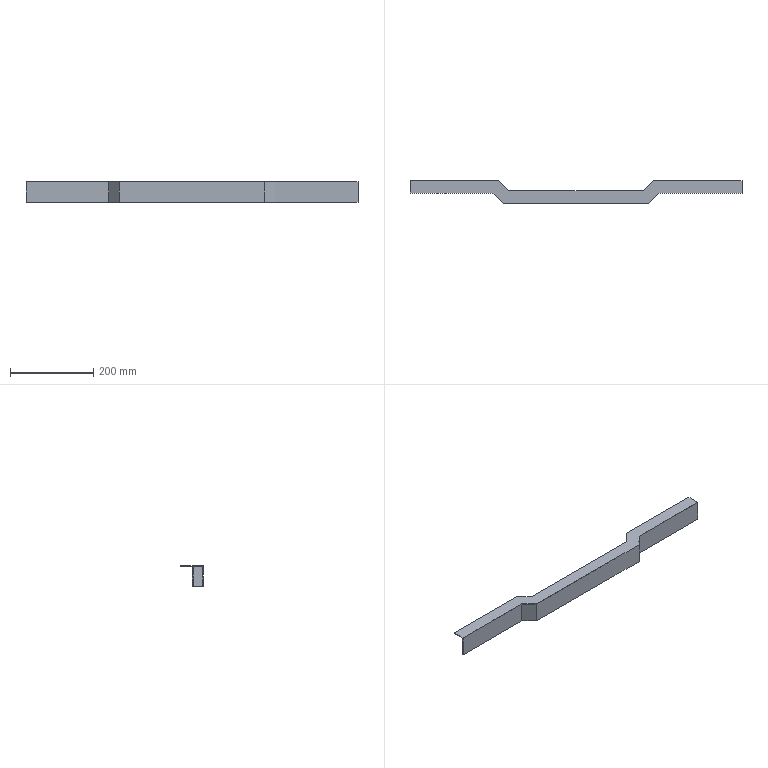Component | SolidWorks | JF21-80.1-1-3(_)-1-SOLID70-1 | 1 solid | 20 faces | box 800 x 55 x 50 mm | volume 128031 mm3 | plane 20
STEP:
#1=CARTESIAN_POINT('',(15.748,-7.677,-5.197));
#2=VERTEX_POINT('',#1);
#3=CARTESIAN_POINT('',(15.748,-7.677,-5.118));
#4=VERTEX_POINT('',#3);
#5=CARTESIAN_POINT('',(15.748,-7.677,-5.118));
#6=DIRECTION('',(0.,0.,1.));
#7=VECTOR('',#6,39.37);
#8=LINE('',#5,#7);
#9=EDGE_CURVE('',#2,#4,#8,.T.);
#10=ORIENTED_EDGE('',*,*,#9,.F.);
#11=CARTESIAN_POINT('',(7.385,-7.677,-5.197));
#12=VERTEX_POINT('',#11);
#13=CARTESIAN_POINT('',(7.385,-7.677,-5.197));
#14=DIRECTION('',(1.,-0.,0.));
#15=VECTOR('',#14,39.37);
#16=LINE('',#13,#15);
#17=EDGE_CURVE('',#12,#2,#16,.T.);
#18=ORIENTED_EDGE('',*,*,#17,.F.);
#19=CARTESIAN_POINT('',(7.385,-7.677,-5.118));
#20=VERTEX_POINT('',#19);
#21=CARTESIAN_POINT('',(7.385,-7.677,-5.118));
#22=DIRECTION('',(0.,0.,-1.));
#23=VECTOR('',#22,39.37);
#24=LINE('',#21,#23);
#25=EDGE_CURVE('',#20,#12,#24,.T.);
#26=ORIENTED_EDGE('',*,*,#25,.F.);
#27=CARTESIAN_POINT('',(7.385,-7.677,-5.118));
#28=DIRECTION('',(1.,-0.,0.));
#29=VECTOR('',#28,39.37);
#30=LINE('',#27,#29);
#31=EDGE_CURVE('',#20,#4,#30,.T.);
#32=ORIENTED_EDGE('',*,*,#31,.T.);
#33=EDGE_LOOP('',(#10,#18,#26,#32));
#34=FACE_OUTER_BOUND('',#33,.T.);
#35=CARTESIAN_POINT('',(7.385,-7.677,-5.118));
#36=DIRECTION('',(-0.,-1.,0.));
#37=DIRECTION('',(-1.,0.,0.));
#38=AXIS2_PLACEMENT_3D('',#35,#36,#37);
#39=PLANE('',#38);
#40=ADVANCED_FACE('',(#34),#39,.F.);
#41=CARTESIAN_POINT('',(15.748,-8.78,-7.087));
#42=VERTEX_POINT('',#41);
#43=CARTESIAN_POINT('',(15.748,-8.78,-5.197));
#44=VERTEX_POINT('',#43);
#45=CARTESIAN_POINT('',(15.748,-8.78,-5.197));
#46=DIRECTION('',(0.,0.,1.));
#47=VECTOR('',#46,39.37);
#48=LINE('',#45,#47);
#49=EDGE_CURVE('',#42,#44,#48,.T.);
#50=ORIENTED_EDGE('',*,*,#49,.F.);
#51=CARTESIAN_POINT('',(7.841,-8.78,-7.087));
#52=VERTEX_POINT('',#51);
#53=CARTESIAN_POINT('',(7.841,-8.78,-7.087));
#54=DIRECTION('',(1.,-0.,0.));
#55=VECTOR('',#54,39.37);
#56=LINE('',#53,#55);
#57=EDGE_CURVE('',#52,#42,#56,.T.);
#58=ORIENTED_EDGE('',*,*,#57,.F.);
#59=CARTESIAN_POINT('',(7.841,-8.78,-5.197));
#60=VERTEX_POINT('',#59);
#61=CARTESIAN_POINT('',(7.841,-8.78,-5.197));
#62=DIRECTION('',(0.,0.,-1.));
#63=VECTOR('',#62,39.37);
#64=LINE('',#61,#63);
#65=EDGE_CURVE('',#60,#52,#64,.T.);
#66=ORIENTED_EDGE('',*,*,#65,.F.);
#67=CARTESIAN_POINT('',(7.841,-8.78,-5.197));
#68=DIRECTION('',(1.,-0.,0.));
#69=VECTOR('',#68,39.37);
#70=LINE('',#67,#69);
#71=EDGE_CURVE('',#60,#44,#70,.T.);
#72=ORIENTED_EDGE('',*,*,#71,.T.);
#73=EDGE_LOOP('',(#50,#58,#66,#72));
#74=FACE_OUTER_BOUND('',#73,.T.);
#75=CARTESIAN_POINT('',(7.841,-8.78,-5.197));
#76=DIRECTION('',(-0.,-1.,0.));
#77=DIRECTION('',(-1.,0.,0.));
#78=AXIS2_PLACEMENT_3D('',#75,#76,#77);
#79=PLANE('',#78);
#80=ADVANCED_FACE('',(#74),#79,.F.);
#81=CARTESIAN_POINT('',(15.748,-8.858,-5.118));
#82=VERTEX_POINT('',#81);
#83=CARTESIAN_POINT('',(15.748,-8.858,-7.087));
#84=VERTEX_POINT('',#83);
#85=CARTESIAN_POINT('',(15.748,-8.858,-7.087));
#86=DIRECTION('',(0.,0.,-1.));
#87=VECTOR('',#86,39.37);
#88=LINE('',#85,#87);
#89=EDGE_CURVE('',#82,#84,#88,.T.);
#90=ORIENTED_EDGE('',*,*,#89,.F.);
#91=CARTESIAN_POINT('',(7.874,-8.858,-5.118));
#92=VERTEX_POINT('',#91);
#93=CARTESIAN_POINT('',(7.874,-8.858,-5.118));
#94=DIRECTION('',(1.,-0.,0.));
#95=VECTOR('',#94,39.37);
#96=LINE('',#93,#95);
#97=EDGE_CURVE('',#92,#82,#96,.T.);
#98=ORIENTED_EDGE('',*,*,#97,.F.);
#99=CARTESIAN_POINT('',(7.874,-8.858,-7.087));
#100=VERTEX_POINT('',#99);
#101=CARTESIAN_POINT('',(7.874,-8.858,-7.087));
#102=DIRECTION('',(0.,0.,1.));
#103=VECTOR('',#102,39.37);
#104=LINE('',#101,#103);
#105=EDGE_CURVE('',#100,#92,#104,.T.);
#106=ORIENTED_EDGE('',*,*,#105,.F.);
#107=CARTESIAN_POINT('',(7.874,-8.858,-7.087));
#108=DIRECTION('',(1.,-0.,0.));
#109=VECTOR('',#108,39.37);
#110=LINE('',#107,#109);
#111=EDGE_CURVE('',#100,#84,#110,.T.);
#112=ORIENTED_EDGE('',*,*,#111,.T.);
#113=EDGE_LOOP('',(#90,#98,#106,#112));
#114=FACE_OUTER_BOUND('',#113,.T.);
#115=CARTESIAN_POINT('',(7.874,-8.858,-7.087));
#116=DIRECTION('',(0.,1.,0.));
#117=DIRECTION('',(1.,-0.,0.));
#118=AXIS2_PLACEMENT_3D('',#115,#116,#117);
#119=PLANE('',#118);
#120=ADVANCED_FACE('',(#114),#119,.F.);
#121=CARTESIAN_POINT('',(6.857,-9.764,-5.197));
#122=VERTEX_POINT('',#121);
#123=CARTESIAN_POINT('',(6.857,-9.764,-5.197));
#124=DIRECTION('',(0.7071,0.7071,0.));
#125=VECTOR('',#124,39.37);
#126=LINE('',#123,#125);
#127=EDGE_CURVE('',#122,#60,#126,.T.);
#128=ORIENTED_EDGE('',*,*,#127,.T.);
#129=ORIENTED_EDGE('',*,*,#65,.T.);
#130=CARTESIAN_POINT('',(6.857,-9.764,-7.087));
#131=VERTEX_POINT('',#130);
#132=CARTESIAN_POINT('',(6.857,-9.764,-7.087));
#133=DIRECTION('',(0.7071,0.7071,0.));
#134=VECTOR('',#133,39.37);
#135=LINE('',#132,#134);
#136=EDGE_CURVE('',#131,#52,#135,.T.);
#137=ORIENTED_EDGE('',*,*,#136,.F.);
#138=CARTESIAN_POINT('',(6.857,-9.764,-5.197));
#139=DIRECTION('',(0.,0.,1.));
#140=VECTOR('',#139,39.37);
#141=LINE('',#138,#140);
#142=EDGE_CURVE('',#131,#122,#141,.T.);
#143=ORIENTED_EDGE('',*,*,#142,.T.);
#144=EDGE_LOOP('',(#128,#129,#137,#143));
#145=FACE_OUTER_BOUND('',#144,.T.);
#146=CARTESIAN_POINT('',(6.857,-9.764,-5.197));
#147=DIRECTION('',(-0.7071,0.7071,0.));
#148=DIRECTION('',(0.7071,0.7071,0.));
#149=AXIS2_PLACEMENT_3D('',#146,#147,#148);
#150=PLANE('',#149);
#151=ADVANCED_FACE('',(#145),#150,.T.);
#152=CARTESIAN_POINT('',(6.89,-9.843,-7.087));
#153=VERTEX_POINT('',#152);
#154=CARTESIAN_POINT('',(6.89,-9.843,-7.087));
#155=DIRECTION('',(0.7071,0.7071,0.));
#156=VECTOR('',#155,39.37);
#157=LINE('',#154,#156);
#158=EDGE_CURVE('',#153,#100,#157,.T.);
#159=ORIENTED_EDGE('',*,*,#158,.T.);
#160=ORIENTED_EDGE('',*,*,#105,.T.);
#161=CARTESIAN_POINT('',(6.89,-9.843,-5.118));
#162=VERTEX_POINT('',#161);
#163=CARTESIAN_POINT('',(6.89,-9.843,-5.118));
#164=DIRECTION('',(0.7071,0.7071,0.));
#165=VECTOR('',#164,39.37);
#166=LINE('',#163,#165);
#167=EDGE_CURVE('',#162,#92,#166,.T.);
#168=ORIENTED_EDGE('',*,*,#167,.F.);
#169=CARTESIAN_POINT('',(6.89,-9.843,-7.087));
#170=DIRECTION('',(0.,0.,-1.));
#171=VECTOR('',#170,39.37);
#172=LINE('',#169,#171);
#173=EDGE_CURVE('',#162,#153,#172,.T.);
#174=ORIENTED_EDGE('',*,*,#173,.T.);
#175=EDGE_LOOP('',(#159,#160,#168,#174));
#176=FACE_OUTER_BOUND('',#175,.T.);
#177=CARTESIAN_POINT('',(6.89,-9.843,-7.087));
#178=DIRECTION('',(0.7071,-0.7071,0.));
#179=DIRECTION('',(-0.7071,-0.7071,0.));
#180=AXIS2_PLACEMENT_3D('',#177,#178,#179);
#181=PLANE('',#180);
#182=ADVANCED_FACE('',(#176),#181,.T.);
#183=CARTESIAN_POINT('',(6.401,-8.661,-5.118));
#184=VERTEX_POINT('',#183);
#185=CARTESIAN_POINT('',(6.401,-8.661,-5.118));
#186=DIRECTION('',(0.7071,0.7071,0.));
#187=VECTOR('',#186,39.37);
#188=LINE('',#185,#187);
#189=EDGE_CURVE('',#184,#20,#188,.T.);
#190=ORIENTED_EDGE('',*,*,#189,.T.);
#191=ORIENTED_EDGE('',*,*,#25,.T.);
#192=CARTESIAN_POINT('',(6.401,-8.661,-5.197));
#193=VERTEX_POINT('',#192);
#194=CARTESIAN_POINT('',(6.401,-8.661,-5.197));
#195=DIRECTION('',(0.7071,0.7071,0.));
#196=VECTOR('',#195,39.37);
#197=LINE('',#194,#196);
#198=EDGE_CURVE('',#193,#12,#197,.T.);
#199=ORIENTED_EDGE('',*,*,#198,.F.);
#200=CARTESIAN_POINT('',(6.401,-8.661,-5.118));
#201=DIRECTION('',(0.,0.,1.));
#202=VECTOR('',#201,39.37);
#203=LINE('',#200,#202);
#204=EDGE_CURVE('',#193,#184,#203,.T.);
#205=ORIENTED_EDGE('',*,*,#204,.T.);
#206=EDGE_LOOP('',(#190,#191,#199,#205));
#207=FACE_OUTER_BOUND('',#206,.T.);
#208=CARTESIAN_POINT('',(6.401,-8.661,-5.118));
#209=DIRECTION('',(-0.7071,0.7071,0.));
#210=DIRECTION('',(0.7071,0.7071,0.));
#211=AXIS2_PLACEMENT_3D('',#208,#209,#210);
#212=PLANE('',#211);
#213=ADVANCED_FACE('',(#207),#212,.T.);
#214=ORIENTED_EDGE('',*,*,#142,.F.);
#215=CARTESIAN_POINT('',(-6.857,-9.764,-7.087));
#216=VERTEX_POINT('',#215);
#217=CARTESIAN_POINT('',(-6.857,-9.764,-7.087));
#218=DIRECTION('',(1.,-0.,0.));
#219=VECTOR('',#218,39.37);
#220=LINE('',#217,#219);
#221=EDGE_CURVE('',#216,#131,#220,.T.);
#222=ORIENTED_EDGE('',*,*,#221,.F.);
#223=CARTESIAN_POINT('',(-6.857,-9.764,-5.197));
#224=VERTEX_POINT('',#223);
#225=CARTESIAN_POINT('',(-6.857,-9.764,-5.197));
#226=DIRECTION('',(0.,0.,-1.));
#227=VECTOR('',#226,39.37);
#228=LINE('',#225,#227);
#229=EDGE_CURVE('',#224,#216,#228,.T.);
#230=ORIENTED_EDGE('',*,*,#229,.F.);
#231=CARTESIAN_POINT('',(-6.857,-9.764,-5.197));
#232=DIRECTION('',(1.,-0.,0.));
#233=VECTOR('',#232,39.37);
#234=LINE('',#231,#233);
#235=EDGE_CURVE('',#224,#122,#234,.T.);
#236=ORIENTED_EDGE('',*,*,#235,.T.);
#237=EDGE_LOOP('',(#214,#222,#230,#236));
#238=FACE_OUTER_BOUND('',#237,.T.);
#239=CARTESIAN_POINT('',(-6.857,-9.764,-5.197));
#240=DIRECTION('',(-0.,-1.,0.));
#241=DIRECTION('',(-1.,0.,0.));
#242=AXIS2_PLACEMENT_3D('',#239,#240,#241);
#243=PLANE('',#242);
#244=ADVANCED_FACE('',(#238),#243,.F.);
#245=ORIENTED_EDGE('',*,*,#173,.F.);
#246=CARTESIAN_POINT('',(-6.89,-9.843,-5.118));
#247=VERTEX_POINT('',#246);
#248=CARTESIAN_POINT('',(-6.89,-9.843,-5.118));
#249=DIRECTION('',(1.,-0.,0.));
#250=VECTOR('',#249,39.37);
#251=LINE('',#248,#250);
#252=EDGE_CURVE('',#247,#162,#251,.T.);
#253=ORIENTED_EDGE('',*,*,#252,.F.);
#254=CARTESIAN_POINT('',(-6.89,-9.843,-7.087));
#255=VERTEX_POINT('',#254);
#256=CARTESIAN_POINT('',(-6.89,-9.843,-7.087));
#257=DIRECTION('',(0.,0.,1.));
#258=VECTOR('',#257,39.37);
#259=LINE('',#256,#258);
#260=EDGE_CURVE('',#255,#247,#259,.T.);
#261=ORIENTED_EDGE('',*,*,#260,.F.);
#262=CARTESIAN_POINT('',(-6.89,-9.843,-7.087));
#263=DIRECTION('',(1.,-0.,0.));
#264=VECTOR('',#263,39.37);
#265=LINE('',#262,#264);
#266=EDGE_CURVE('',#255,#153,#265,.T.);
#267=ORIENTED_EDGE('',*,*,#266,.T.);
#268=EDGE_LOOP('',(#245,#253,#261,#267));
#269=FACE_OUTER_BOUND('',#268,.T.);
#270=CARTESIAN_POINT('',(-6.89,-9.843,-7.087));
#271=DIRECTION('',(0.,1.,0.));
#272=DIRECTION('',(1.,-0.,0.));
#273=AXIS2_PLACEMENT_3D('',#270,#271,#272);
#274=PLANE('',#273);
#275=ADVANCED_FACE('',(#269),#274,.F.);
#276=ORIENTED_EDGE('',*,*,#204,.F.);
#277=CARTESIAN_POINT('',(-6.401,-8.661,-5.197));
#278=VERTEX_POINT('',#277);
#279=CARTESIAN_POINT('',(-6.401,-8.661,-5.197));
#280=DIRECTION('',(1.,-0.,0.));
#281=VECTOR('',#280,39.37);
#282=LINE('',#279,#281);
#283=EDGE_CURVE('',#278,#193,#282,.T.);
#284=ORIENTED_EDGE('',*,*,#283,.F.);
#285=CARTESIAN_POINT('',(-6.401,-8.661,-5.118));
#286=VERTEX_POINT('',#285);
#287=CARTESIAN_POINT('',(-6.401,-8.661,-5.118));
#288=DIRECTION('',(0.,0.,-1.));
#289=VECTOR('',#288,39.37);
#290=LINE('',#287,#289);
#291=EDGE_CURVE('',#286,#278,#290,.T.);
#292=ORIENTED_EDGE('',*,*,#291,.F.);
#293=CARTESIAN_POINT('',(-6.401,-8.661,-5.118));
#294=DIRECTION('',(1.,-0.,0.));
#295=VECTOR('',#294,39.37);
#296=LINE('',#293,#295);
#297=EDGE_CURVE('',#286,#184,#296,.T.);
#298=ORIENTED_EDGE('',*,*,#297,.T.);
#299=EDGE_LOOP('',(#276,#284,#292,#298));
#300=FACE_OUTER_BOUND('',#299,.T.);
#301=CARTESIAN_POINT('',(-6.401,-8.661,-5.118));
#302=DIRECTION('',(-0.,-1.,0.));
#303=DIRECTION('',(-1.,0.,0.));
#304=AXIS2_PLACEMENT_3D('',#301,#302,#303);
#305=PLANE('',#304);
#306=ADVANCED_FACE('',(#300),#305,.F.);
#307=CARTESIAN_POINT('',(-7.841,-8.78,-5.197));
#308=VERTEX_POINT('',#307);
#309=CARTESIAN_POINT('',(-7.841,-8.78,-5.197));
#310=DIRECTION('',(0.7071,-0.7071,0.));
#311=VECTOR('',#310,39.37);
#312=LINE('',#309,#311);
#313=EDGE_CURVE('',#308,#224,#312,.T.);
#314=ORIENTED_EDGE('',*,*,#313,.T.);
#315=ORIENTED_EDGE('',*,*,#229,.T.);
#316=CARTESIAN_POINT('',(-7.841,-8.78,-7.087));
#317=VERTEX_POINT('',#316);
#318=CARTESIAN_POINT('',(-7.841,-8.78,-7.087));
#319=DIRECTION('',(0.7071,-0.7071,0.));
#320=VECTOR('',#319,39.37);
#321=LINE('',#318,#320);
#322=EDGE_CURVE('',#317,#216,#321,.T.);
#323=ORIENTED_EDGE('',*,*,#322,.F.);
#324=CARTESIAN_POINT('',(-7.841,-8.78,-5.197));
#325=DIRECTION('',(0.,0.,1.));
#326=VECTOR('',#325,39.37);
#327=LINE('',#324,#326);
#328=EDGE_CURVE('',#317,#308,#327,.T.);
#329=ORIENTED_EDGE('',*,*,#328,.T.);
#330=EDGE_LOOP('',(#314,#315,#323,#329));
#331=FACE_OUTER_BOUND('',#330,.T.);
#332=CARTESIAN_POINT('',(-7.841,-8.78,-5.197));
#333=DIRECTION('',(0.7071,0.7071,0.));
#334=DIRECTION('',(0.7071,-0.7071,0.));
#335=AXIS2_PLACEMENT_3D('',#332,#333,#334);
#336=PLANE('',#335);
#337=ADVANCED_FACE('',(#331),#336,.T.);
#338=CARTESIAN_POINT('',(-7.874,-8.858,-7.087));
#339=VERTEX_POINT('',#338);
#340=CARTESIAN_POINT('',(-7.874,-8.858,-7.087));
#341=DIRECTION('',(0.7071,-0.7071,0.));
#342=VECTOR('',#341,39.37);
#343=LINE('',#340,#342);
#344=EDGE_CURVE('',#339,#255,#343,.T.);
#345=ORIENTED_EDGE('',*,*,#344,.T.);
#346=ORIENTED_EDGE('',*,*,#260,.T.);
#347=CARTESIAN_POINT('',(-7.874,-8.858,-5.118));
#348=VERTEX_POINT('',#347);
#349=CARTESIAN_POINT('',(-7.874,-8.858,-5.118));
#350=DIRECTION('',(0.7071,-0.7071,0.));
#351=VECTOR('',#350,39.37);
#352=LINE('',#349,#351);
#353=EDGE_CURVE('',#348,#247,#352,.T.);
#354=ORIENTED_EDGE('',*,*,#353,.F.);
#355=CARTESIAN_POINT('',(-7.874,-8.858,-7.087));
#356=DIRECTION('',(0.,0.,-1.));
#357=VECTOR('',#356,39.37);
#358=LINE('',#355,#357);
#359=EDGE_CURVE('',#348,#339,#358,.T.);
#360=ORIENTED_EDGE('',*,*,#359,.T.);
#361=EDGE_LOOP('',(#345,#346,#354,#360));
#362=FACE_OUTER_BOUND('',#361,.T.);
#363=CARTESIAN_POINT('',(-7.874,-8.858,-7.087));
#364=DIRECTION('',(-0.7071,-0.7071,0.));
#365=DIRECTION('',(-0.7071,0.7071,0.));
#366=AXIS2_PLACEMENT_3D('',#363,#364,#365);
#367=PLANE('',#366);
#368=ADVANCED_FACE('',(#362),#367,.T.);
#369=CARTESIAN_POINT('',(-7.385,-7.677,-5.118));
#370=VERTEX_POINT('',#369);
#371=CARTESIAN_POINT('',(-7.385,-7.677,-5.118));
#372=DIRECTION('',(0.7071,-0.7071,0.));
#373=VECTOR('',#372,39.37);
#374=LINE('',#371,#373);
#375=EDGE_CURVE('',#370,#286,#374,.T.);
#376=ORIENTED_EDGE('',*,*,#375,.T.);
#377=ORIENTED_EDGE('',*,*,#291,.T.);
#378=CARTESIAN_POINT('',(-7.385,-7.677,-5.197));
#379=VERTEX_POINT('',#378);
#380=CARTESIAN_POINT('',(-7.385,-7.677,-5.197));
#381=DIRECTION('',(0.7071,-0.7071,0.));
#382=VECTOR('',#381,39.37);
#383=LINE('',#380,#382);
#384=EDGE_CURVE('',#379,#278,#383,.T.);
#385=ORIENTED_EDGE('',*,*,#384,.F.);
#386=CARTESIAN_POINT('',(-7.385,-7.677,-5.118));
#387=DIRECTION('',(0.,0.,1.));
#388=VECTOR('',#387,39.37);
#389=LINE('',#386,#388);
#390=EDGE_CURVE('',#379,#370,#389,.T.);
#391=ORIENTED_EDGE('',*,*,#390,.T.);
#392=EDGE_LOOP('',(#376,#377,#385,#391));
#393=FACE_OUTER_BOUND('',#392,.T.);
#394=CARTESIAN_POINT('',(-7.385,-7.677,-5.118));
#395=DIRECTION('',(0.7071,0.7071,0.));
#396=DIRECTION('',(0.7071,-0.7071,0.));
#397=AXIS2_PLACEMENT_3D('',#394,#395,#396);
#398=PLANE('',#397);
#399=ADVANCED_FACE('',(#393),#398,.T.);
#400=ORIENTED_EDGE('',*,*,#328,.F.);
#401=CARTESIAN_POINT('',(-15.748,-8.78,-7.087));
#402=VERTEX_POINT('',#401);
#403=CARTESIAN_POINT('',(-5.334,-8.78,-7.087));
#404=DIRECTION('',(-1.,-0.,0.));
#405=VECTOR('',#404,39.37);
#406=LINE('',#403,#405);
#407=EDGE_CURVE('',#317,#402,#406,.T.);
#408=ORIENTED_EDGE('',*,*,#407,.T.);
#409=CARTESIAN_POINT('',(-15.748,-8.78,-5.197));
#410=VERTEX_POINT('',#409);
#411=CARTESIAN_POINT('',(-15.748,-8.78,-5.197));
#412=DIRECTION('',(0.,0.,1.));
#413=VECTOR('',#412,39.37);
#414=LINE('',#411,#413);
#415=EDGE_CURVE('',#402,#410,#414,.T.);
#416=ORIENTED_EDGE('',*,*,#415,.T.);
#417=CARTESIAN_POINT('',(-5.334,-8.78,-5.197));
#418=DIRECTION('',(-1.,-0.,0.));
#419=VECTOR('',#418,39.37);
#420=LINE('',#417,#419);
#421=EDGE_CURVE('',#308,#410,#420,.T.);
#422=ORIENTED_EDGE('',*,*,#421,.F.);
#423=EDGE_LOOP('',(#400,#408,#416,#422));
#424=FACE_OUTER_BOUND('',#423,.T.);
#425=CARTESIAN_POINT('',(-5.334,-8.78,-5.197));
#426=DIRECTION('',(0.,-1.,0.));
#427=DIRECTION('',(-1.,-0.,0.));
#428=AXIS2_PLACEMENT_3D('',#425,#426,#427);
#429=PLANE('',#428);
#430=ADVANCED_FACE('',(#424),#429,.F.);
#431=CARTESIAN_POINT('',(-15.748,-7.677,-5.197));
#432=VERTEX_POINT('',#431);
#433=CARTESIAN_POINT('',(-5.334,-7.677,-5.197));
#434=DIRECTION('',(-1.,-0.,0.));
#435=VECTOR('',#434,39.37);
#436=LINE('',#433,#435);
#437=EDGE_CURVE('',#379,#432,#436,.T.);
#438=ORIENTED_EDGE('',*,*,#437,.F.);
#439=ORIENTED_EDGE('',*,*,#384,.T.);
#440=ORIENTED_EDGE('',*,*,#283,.T.);
#441=ORIENTED_EDGE('',*,*,#198,.T.);
#442=ORIENTED_EDGE('',*,*,#17,.T.);
#443=CARTESIAN_POINT('',(15.748,-2.783,-5.197));
#444=DIRECTION('',(0.,1.,0.));
#445=VECTOR('',#444,39.37);
#446=LINE('',#443,#445);
#447=EDGE_CURVE('',#44,#2,#446,.T.);
#448=ORIENTED_EDGE('',*,*,#447,.F.);
#449=ORIENTED_EDGE('',*,*,#71,.F.);
#450=ORIENTED_EDGE('',*,*,#127,.F.);
#451=ORIENTED_EDGE('',*,*,#235,.F.);
#452=ORIENTED_EDGE('',*,*,#313,.F.);
#453=ORIENTED_EDGE('',*,*,#421,.T.);
#454=CARTESIAN_POINT('',(-15.748,-7.677,-5.197));
#455=DIRECTION('',(0.,1.,0.));
#456=VECTOR('',#455,39.37);
#457=LINE('',#454,#456);
#458=EDGE_CURVE('',#410,#432,#457,.T.);
#459=ORIENTED_EDGE('',*,*,#458,.T.);
#460=EDGE_LOOP('',(#438,#439,#440,#441,#442,#448,#449,#450,#451,#452,#453,#459));
#461=FACE_OUTER_BOUND('',#460,.T.);
#462=CARTESIAN_POINT('',(-5.334,-7.677,-5.197));
#463=DIRECTION('',(0.,0.,1.));
#464=DIRECTION('',(-1.,0.,0.));
#465=AXIS2_PLACEMENT_3D('',#462,#463,#464);
#466=PLANE('',#465);
#467=ADVANCED_FACE('',(#461),#466,.F.);
#468=ORIENTED_EDGE('',*,*,#390,.F.);
#469=ORIENTED_EDGE('',*,*,#437,.T.);
#470=CARTESIAN_POINT('',(-15.748,-7.677,-5.118));
#471=VERTEX_POINT('',#470);
#472=CARTESIAN_POINT('',(-15.748,-7.677,-5.118));
#473=DIRECTION('',(0.,0.,1.));
#474=VECTOR('',#473,39.37);
#475=LINE('',#472,#474);
#476=EDGE_CURVE('',#432,#471,#475,.T.);
#477=ORIENTED_EDGE('',*,*,#476,.T.);
#478=CARTESIAN_POINT('',(-5.334,-7.677,-5.118));
#479=DIRECTION('',(-1.,-0.,0.));
#480=VECTOR('',#479,39.37);
#481=LINE('',#478,#480);
#482=EDGE_CURVE('',#370,#471,#481,.T.);
#483=ORIENTED_EDGE('',*,*,#482,.F.);
#484=EDGE_LOOP('',(#468,#469,#477,#483));
#485=FACE_OUTER_BOUND('',#484,.T.);
#486=CARTESIAN_POINT('',(-5.334,-7.677,-5.118));
#487=DIRECTION('',(0.,-1.,0.));
#488=DIRECTION('',(-1.,-0.,0.));
#489=AXIS2_PLACEMENT_3D('',#486,#487,#488);
#490=PLANE('',#489);
#491=ADVANCED_FACE('',(#485),#490,.F.);
#492=CARTESIAN_POINT('',(-15.748,-8.858,-5.118));
#493=VERTEX_POINT('',#492);
#494=CARTESIAN_POINT('',(-5.334,-8.858,-5.118));
#495=DIRECTION('',(-1.,-0.,0.));
#496=VECTOR('',#495,39.37);
#497=LINE('',#494,#496);
#498=EDGE_CURVE('',#348,#493,#497,.T.);
#499=ORIENTED_EDGE('',*,*,#498,.F.);
#500=ORIENTED_EDGE('',*,*,#353,.T.);
#501=ORIENTED_EDGE('',*,*,#252,.T.);
#502=ORIENTED_EDGE('',*,*,#167,.T.);
#503=ORIENTED_EDGE('',*,*,#97,.T.);
#504=CARTESIAN_POINT('',(15.748,-3.496,-5.118));
#505=DIRECTION('',(-0.,-1.,0.));
#506=VECTOR('',#505,39.37);
#507=LINE('',#504,#506);
#508=EDGE_CURVE('',#4,#82,#507,.T.);
#509=ORIENTED_EDGE('',*,*,#508,.F.);
#510=ORIENTED_EDGE('',*,*,#31,.F.);
#511=ORIENTED_EDGE('',*,*,#189,.F.);
#512=ORIENTED_EDGE('',*,*,#297,.F.);
#513=ORIENTED_EDGE('',*,*,#375,.F.);
#514=ORIENTED_EDGE('',*,*,#482,.T.);
#515=CARTESIAN_POINT('',(-15.748,-8.858,-5.118));
#516=DIRECTION('',(0.,-1.,0.));
#517=VECTOR('',#516,39.37);
#518=LINE('',#515,#517);
#519=EDGE_CURVE('',#471,#493,#518,.T.);
#520=ORIENTED_EDGE('',*,*,#519,.T.);
#521=EDGE_LOOP('',(#499,#500,#501,#502,#503,#509,#510,#511,#512,#513,#514,#520));
#522=FACE_OUTER_BOUND('',#521,.T.);
#523=CARTESIAN_POINT('',(-5.334,-8.858,-5.118));
#524=DIRECTION('',(0.,0.,-1.));
#525=DIRECTION('',(1.,0.,0.));
#526=AXIS2_PLACEMENT_3D('',#523,#524,#525);
#527=PLANE('',#526);
#528=ADVANCED_FACE('',(#522),#527,.F.);
#529=ORIENTED_EDGE('',*,*,#359,.F.);
#530=ORIENTED_EDGE('',*,*,#498,.T.);
#531=CARTESIAN_POINT('',(-15.748,-8.858,-7.087));
#532=VERTEX_POINT('',#531);
#533=CARTESIAN_POINT('',(-15.748,-8.858,-7.087));
#534=DIRECTION('',(0.,0.,-1.));
#535=VECTOR('',#534,39.37);
#536=LINE('',#533,#535);
#537=EDGE_CURVE('',#493,#532,#536,.T.);
#538=ORIENTED_EDGE('',*,*,#537,.T.);
#539=CARTESIAN_POINT('',(-5.334,-8.858,-7.087));
#540=DIRECTION('',(-1.,-0.,0.));
#541=VECTOR('',#540,39.37);
#542=LINE('',#539,#541);
#543=EDGE_CURVE('',#339,#532,#542,.T.);
#544=ORIENTED_EDGE('',*,*,#543,.F.);
#545=EDGE_LOOP('',(#529,#530,#538,#544));
#546=FACE_OUTER_BOUND('',#545,.T.);
#547=CARTESIAN_POINT('',(-5.334,-8.858,-7.087));
#548=DIRECTION('',(-0.,1.,0.));
#549=DIRECTION('',(1.,0.,0.));
#550=AXIS2_PLACEMENT_3D('',#547,#548,#549);
#551=PLANE('',#550);
#552=ADVANCED_FACE('',(#546),#551,.F.);
#553=ORIENTED_EDGE('',*,*,#407,.F.);
#554=ORIENTED_EDGE('',*,*,#322,.T.);
#555=ORIENTED_EDGE('',*,*,#221,.T.);
#556=ORIENTED_EDGE('',*,*,#136,.T.);
#557=ORIENTED_EDGE('',*,*,#57,.T.);
#558=CARTESIAN_POINT('',(15.748,-3.448,-7.087));
#559=DIRECTION('',(0.,1.,-0.));
#560=VECTOR('',#559,39.37);
#561=LINE('',#558,#560);
#562=EDGE_CURVE('',#84,#42,#561,.T.);
#563=ORIENTED_EDGE('',*,*,#562,.F.);
#564=ORIENTED_EDGE('',*,*,#111,.F.);
#565=ORIENTED_EDGE('',*,*,#158,.F.);
#566=ORIENTED_EDGE('',*,*,#266,.F.);
#567=ORIENTED_EDGE('',*,*,#344,.F.);
#568=ORIENTED_EDGE('',*,*,#543,.T.);
#569=CARTESIAN_POINT('',(-15.748,-8.78,-7.087));
#570=DIRECTION('',(0.,1.,-0.));
#571=VECTOR('',#570,39.37);
#572=LINE('',#569,#571);
#573=EDGE_CURVE('',#532,#402,#572,.T.);
#574=ORIENTED_EDGE('',*,*,#573,.T.);
#575=EDGE_LOOP('',(#553,#554,#555,#556,#557,#563,#564,#565,#566,#567,#568,#574));
#576=FACE_OUTER_BOUND('',#575,.T.);
#577=CARTESIAN_POINT('',(-5.334,-8.78,-7.087));
#578=DIRECTION('',(-0.,0.,1.));
#579=DIRECTION('',(0.,1.,-0.));
#580=AXIS2_PLACEMENT_3D('',#577,#578,#579);
#581=PLANE('',#580);
#582=ADVANCED_FACE('',(#576),#581,.F.);
#583=ORIENTED_EDGE('',*,*,#573,.F.);
#584=ORIENTED_EDGE('',*,*,#537,.F.);
#585=ORIENTED_EDGE('',*,*,#519,.F.);
#586=ORIENTED_EDGE('',*,*,#476,.F.);
#587=ORIENTED_EDGE('',*,*,#458,.F.);
#588=ORIENTED_EDGE('',*,*,#415,.F.);
#589=EDGE_LOOP('',(#583,#584,#585,#586,#587,#588));
#590=FACE_OUTER_BOUND('',#589,.T.);
#591=CARTESIAN_POINT('',(-15.748,-8.858,-7.087));
#592=DIRECTION('',(-1.,0.,0.));
#593=DIRECTION('',(0.,0.,-1.));
#594=AXIS2_PLACEMENT_3D('',#591,#592,#593);
#595=PLANE('',#594);
#596=ADVANCED_FACE('',(#590),#595,.T.);
#597=ORIENTED_EDGE('',*,*,#9,.T.);
#598=ORIENTED_EDGE('',*,*,#508,.T.);
#599=ORIENTED_EDGE('',*,*,#89,.T.);
#600=ORIENTED_EDGE('',*,*,#562,.T.);
#601=ORIENTED_EDGE('',*,*,#49,.T.);
#602=ORIENTED_EDGE('',*,*,#447,.T.);
#603=EDGE_LOOP('',(#597,#598,#599,#600,#601,#602));
#604=FACE_OUTER_BOUND('',#603,.T.);
#605=CARTESIAN_POINT('',(15.748,-8.268,-6.102));
#606=DIRECTION('',(1.,-0.,0.));
#607=DIRECTION('',(-0.,-1.,0.));
#608=AXIS2_PLACEMENT_3D('',#605,#606,#607);
#609=PLANE('',#608);
#610=ADVANCED_FACE('',(#604),#609,.T.);
#611=CLOSED_SHELL('',(#40,#80,#120,#151,#182,#213,#244,#275,#306,#337,#368,#399,#430,#467,#491,#528,#552,#582,#596,#610));
#612=MANIFOLD_SOLID_BREP('',#611);
#613=CARTESIAN_POINT('',(0.,0.,0.));
#614=DIRECTION('',(0.,0.,1.));
#615=DIRECTION('',(1.,0.,0.));
#616=AXIS2_PLACEMENT_3D('',#613,#614,#615);
#617=(LENGTH_UNIT()NAMED_UNIT(*)SI_UNIT($,.METRE.));
#618=LENGTH_MEASURE_WITH_UNIT(LENGTH_MEASURE(0.0254),#617);
#619=DIMENSIONAL_EXPONENTS(1.,0.,0.,0.,0.,0.,0.);
#620=(CONVERSION_BASED_UNIT('',#618)LENGTH_UNIT()NAMED_UNIT(#619));
#621=UNCERTAINTY_MEASURE_WITH_UNIT(LENGTH_MEASURE(0.00001),#620,'','');
#622=(NAMED_UNIT(*)PLANE_ANGLE_UNIT()SI_UNIT($,.RADIAN.));
#623=(NAMED_UNIT(*)SI_UNIT($,.STERADIAN.)SOLID_ANGLE_UNIT());
#624=(GEOMETRIC_REPRESENTATION_CONTEXT(3)GLOBAL_UNCERTAINTY_ASSIGNED_CONTEXT((#621))GLOBAL_UNIT_ASSIGNED_CONTEXT((#620,#622,#623))REPRESENTATION_CONTEXT('',''));
#625=ADVANCED_BREP_SHAPE_REPRESENTATION('',(#612,#616),#624);
#626=COLOUR_RGB('',0.7922,0.8196,0.9333);
#627=FILL_AREA_STYLE_COLOUR('',#626);
#628=FILL_AREA_STYLE('',(#627));
#629=SURFACE_STYLE_FILL_AREA(#628);
#630=SURFACE_SIDE_STYLE('',(#629));
#631=SURFACE_STYLE_USAGE(.BOTH.,#630);
#632=PRESENTATION_STYLE_ASSIGNMENT((#631));
#633=STYLED_ITEM('',(#632),#612);
#634=PRESENTATION_LAYER_ASSIGNMENT('','',(#633));
#635=(LENGTH_UNIT()NAMED_UNIT(*)SI_UNIT($,.METRE.));
#636=LENGTH_MEASURE_WITH_UNIT(LENGTH_MEASURE(0.0254),#635);
#637=DIMENSIONAL_EXPONENTS(1.,0.,0.,0.,0.,0.,0.);
#638=(CONVERSION_BASED_UNIT('',#636)LENGTH_UNIT()NAMED_UNIT(#637));
#639=UNCERTAINTY_MEASURE_WITH_UNIT(LENGTH_MEASURE(0.00001),#638,'','');
#640=(NAMED_UNIT(*)PLANE_ANGLE_UNIT()SI_UNIT($,.RADIAN.));
#641=(NAMED_UNIT(*)SI_UNIT($,.STERADIAN.)SOLID_ANGLE_UNIT());
#642=(GEOMETRIC_REPRESENTATION_CONTEXT(3)GLOBAL_UNCERTAINTY_ASSIGNED_CONTEXT((#639))GLOBAL_UNIT_ASSIGNED_CONTEXT((#638,#640,#641))REPRESENTATION_CONTEXT('',''));
#643=MECHANICAL_DESIGN_GEOMETRIC_PRESENTATION_REPRESENTATION('',(#633),#642);